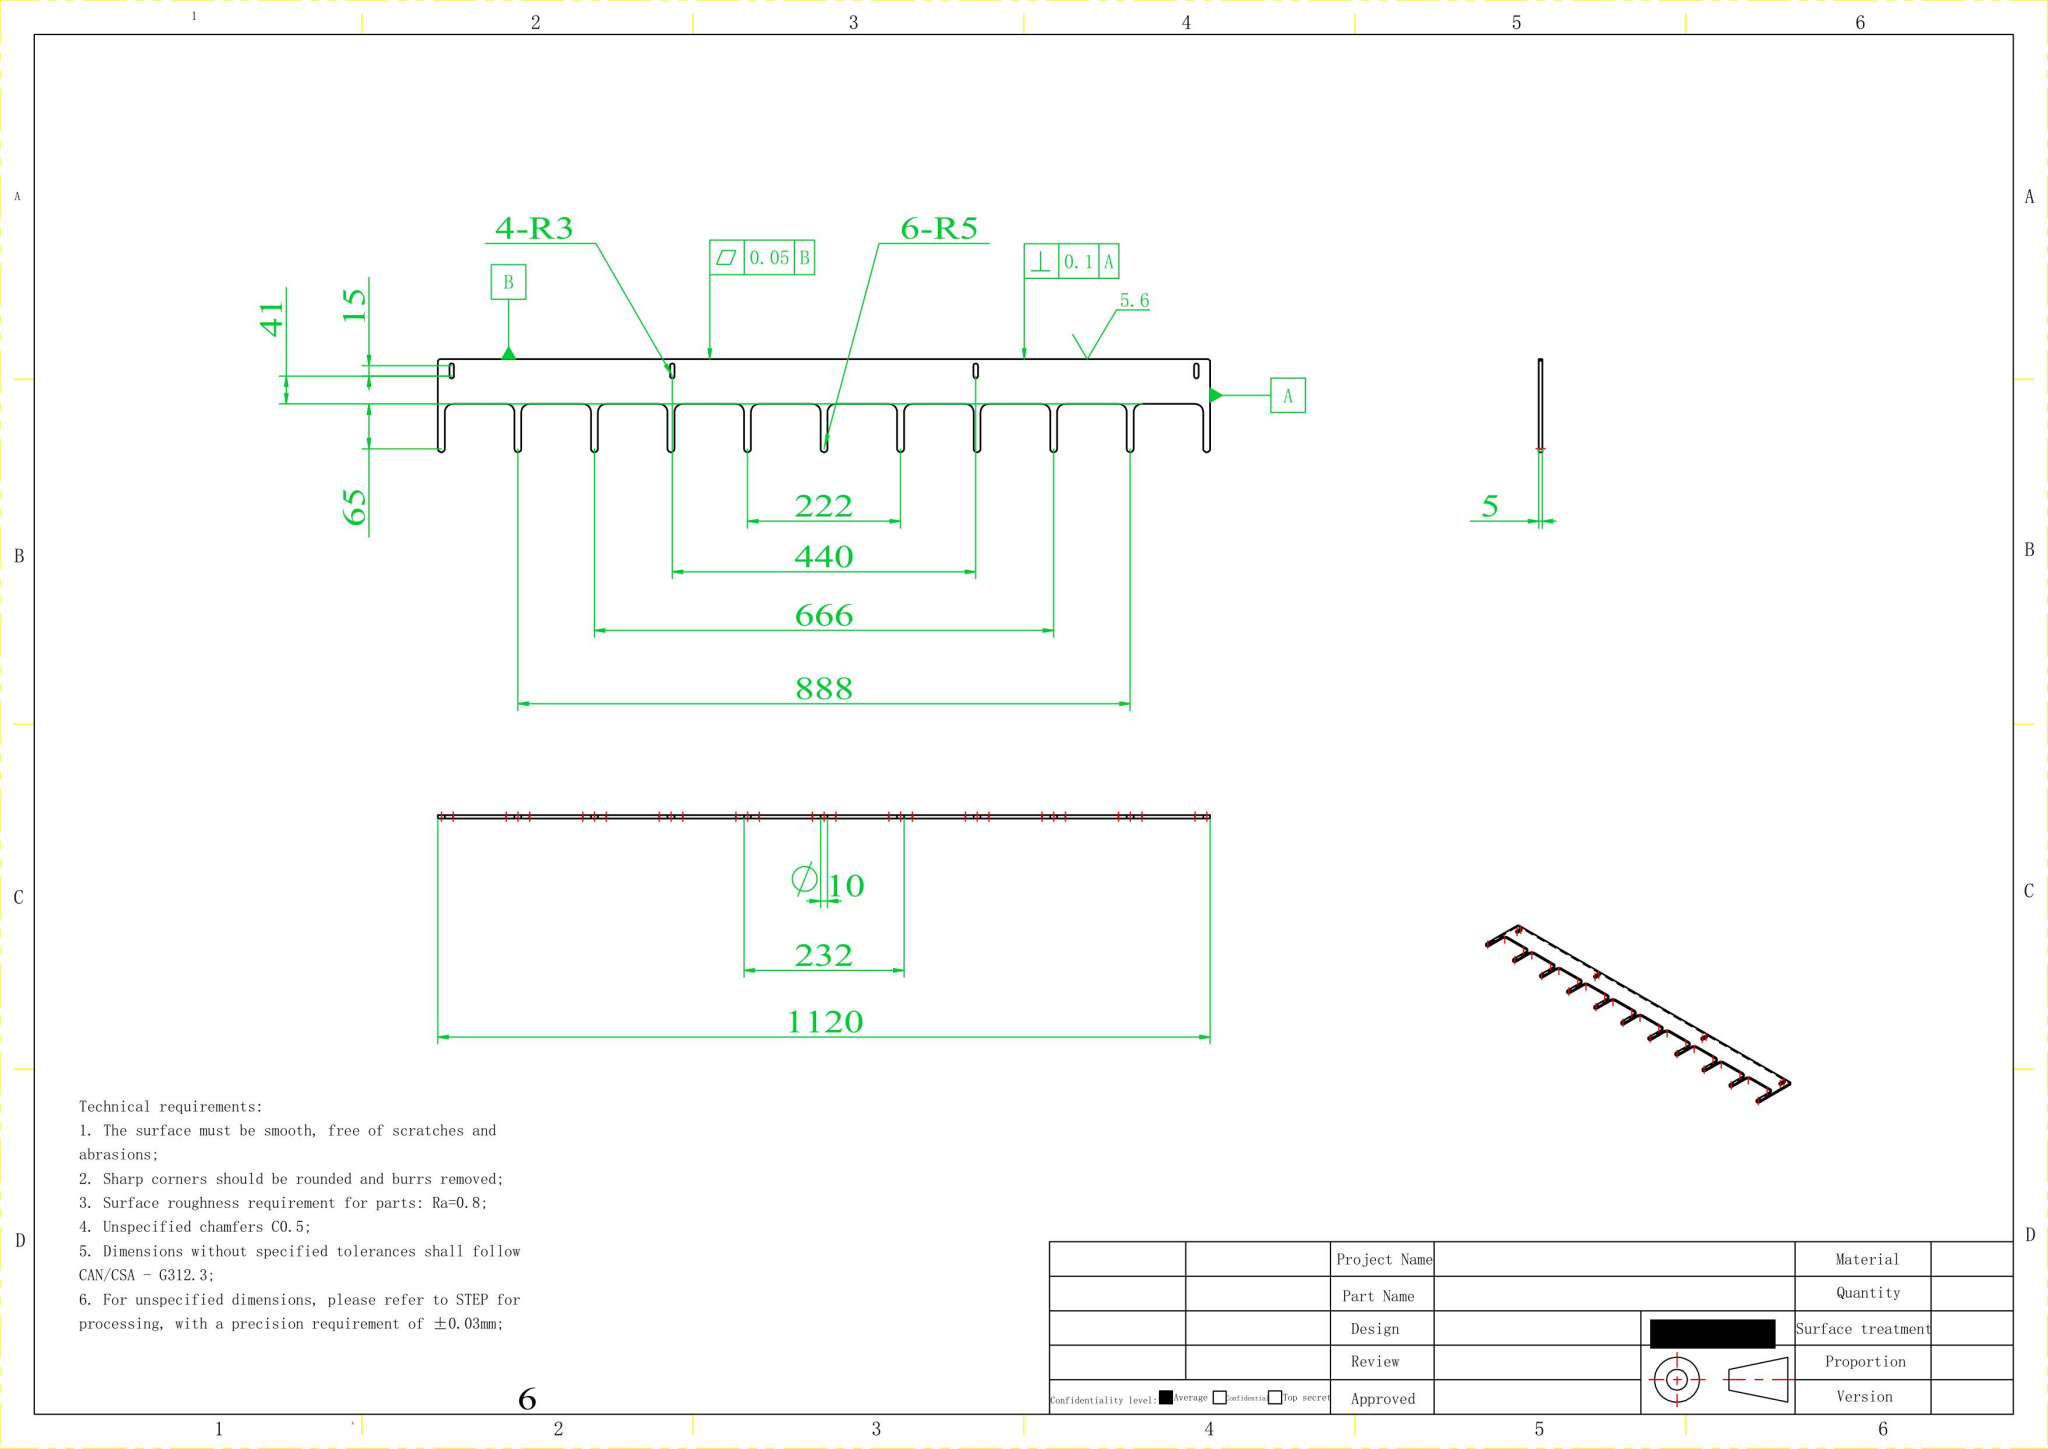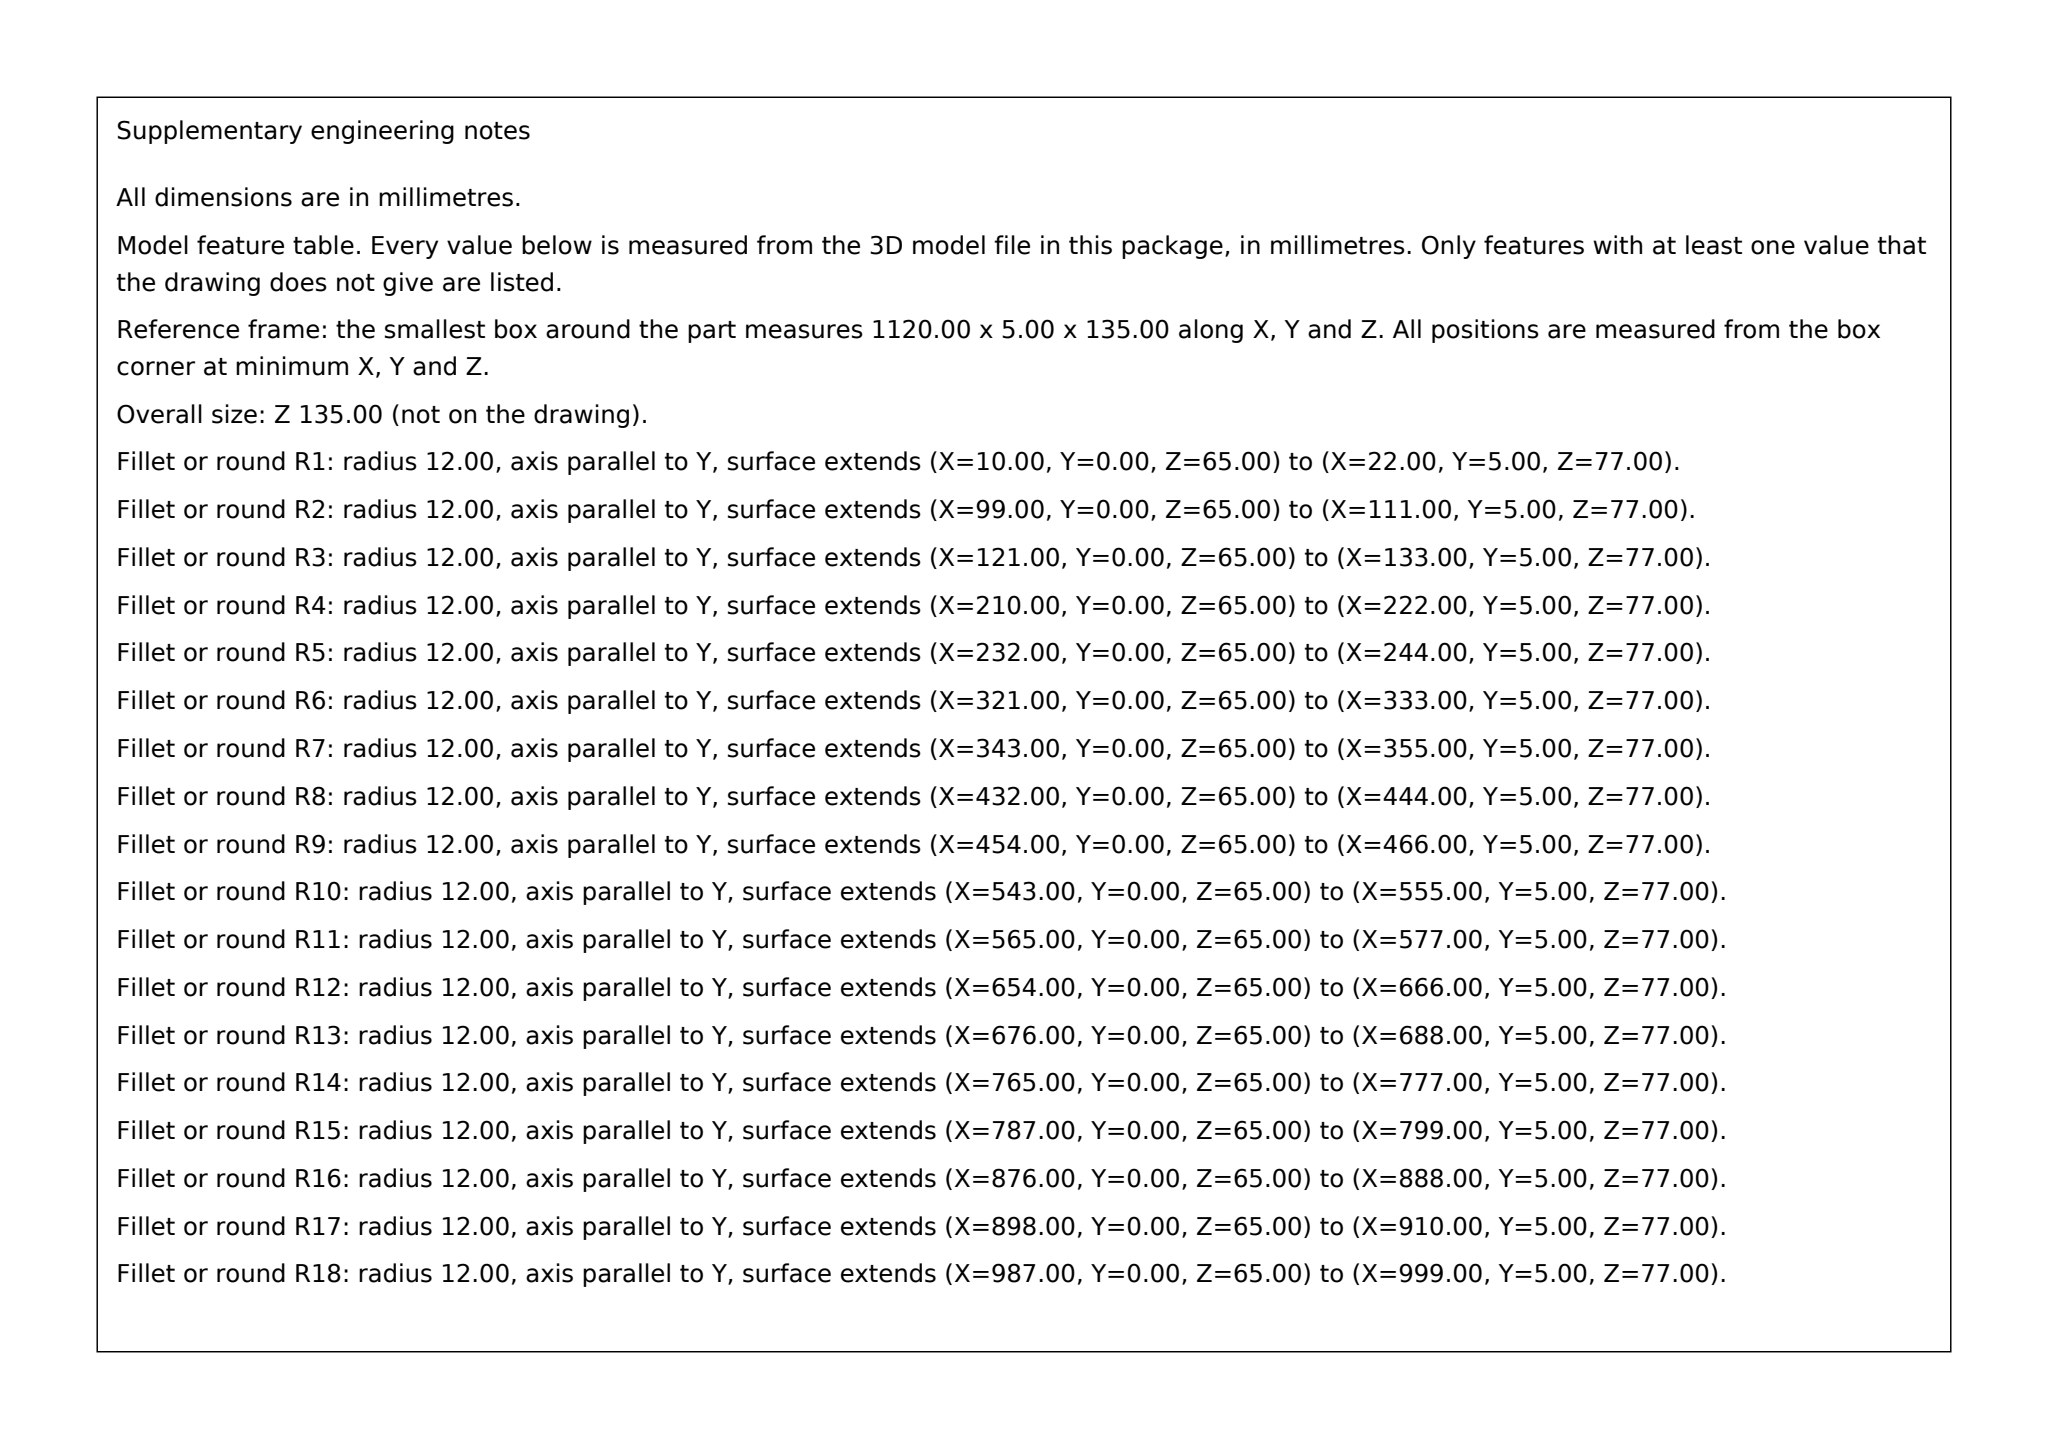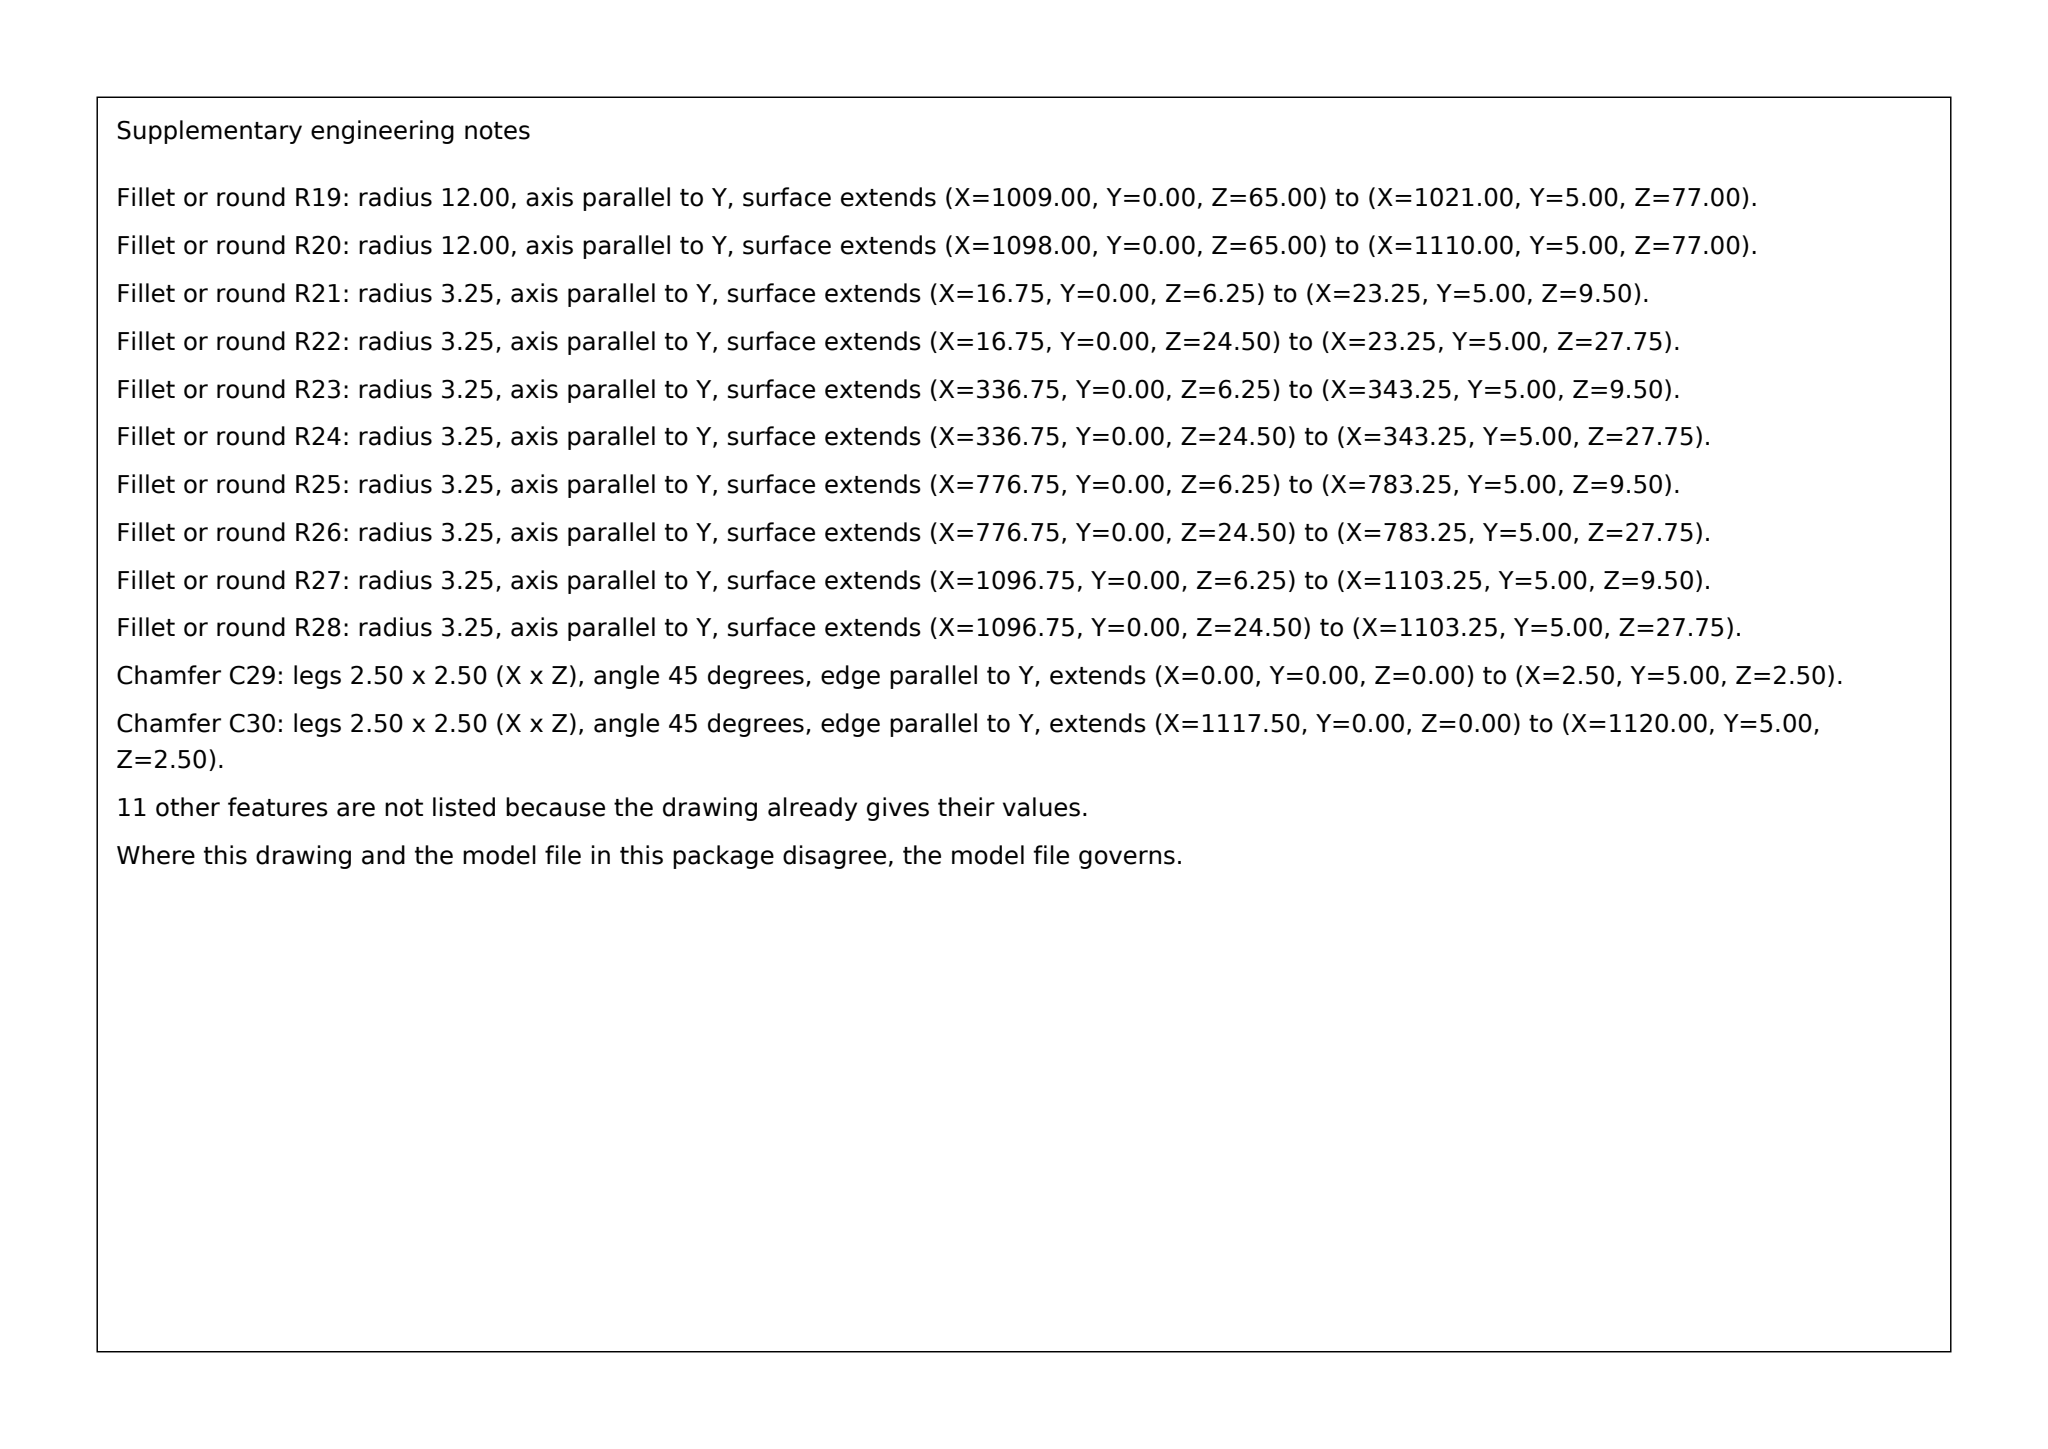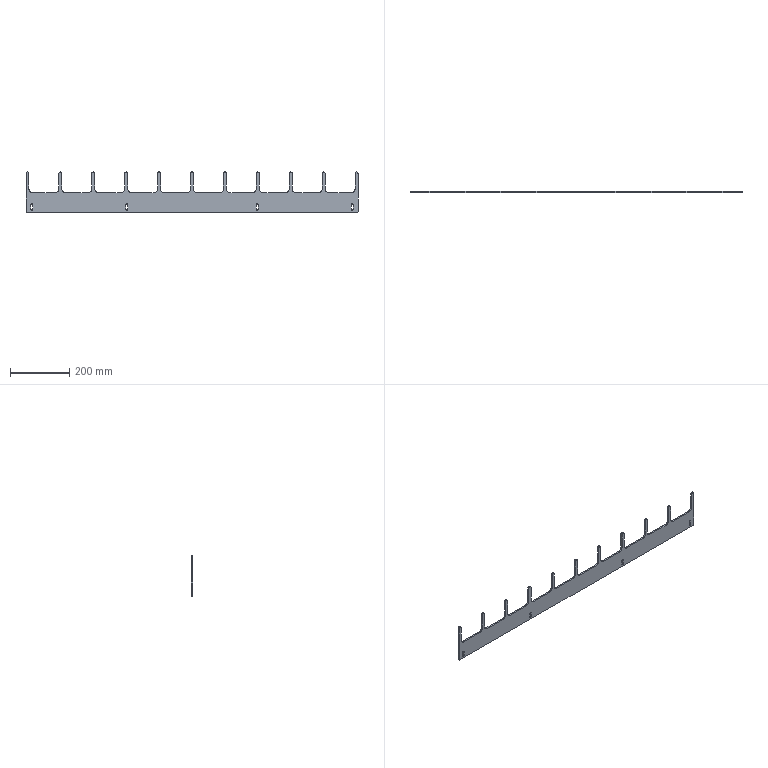Part | SolidWorks | mm | 1 solid | 84 faces | box 1120 x 5 x 135 mm | volume 402355 mm3 | plane 45 | cylinder 39 | commonest cylinder face diameters 24 x20 10 x11 6.5 x8